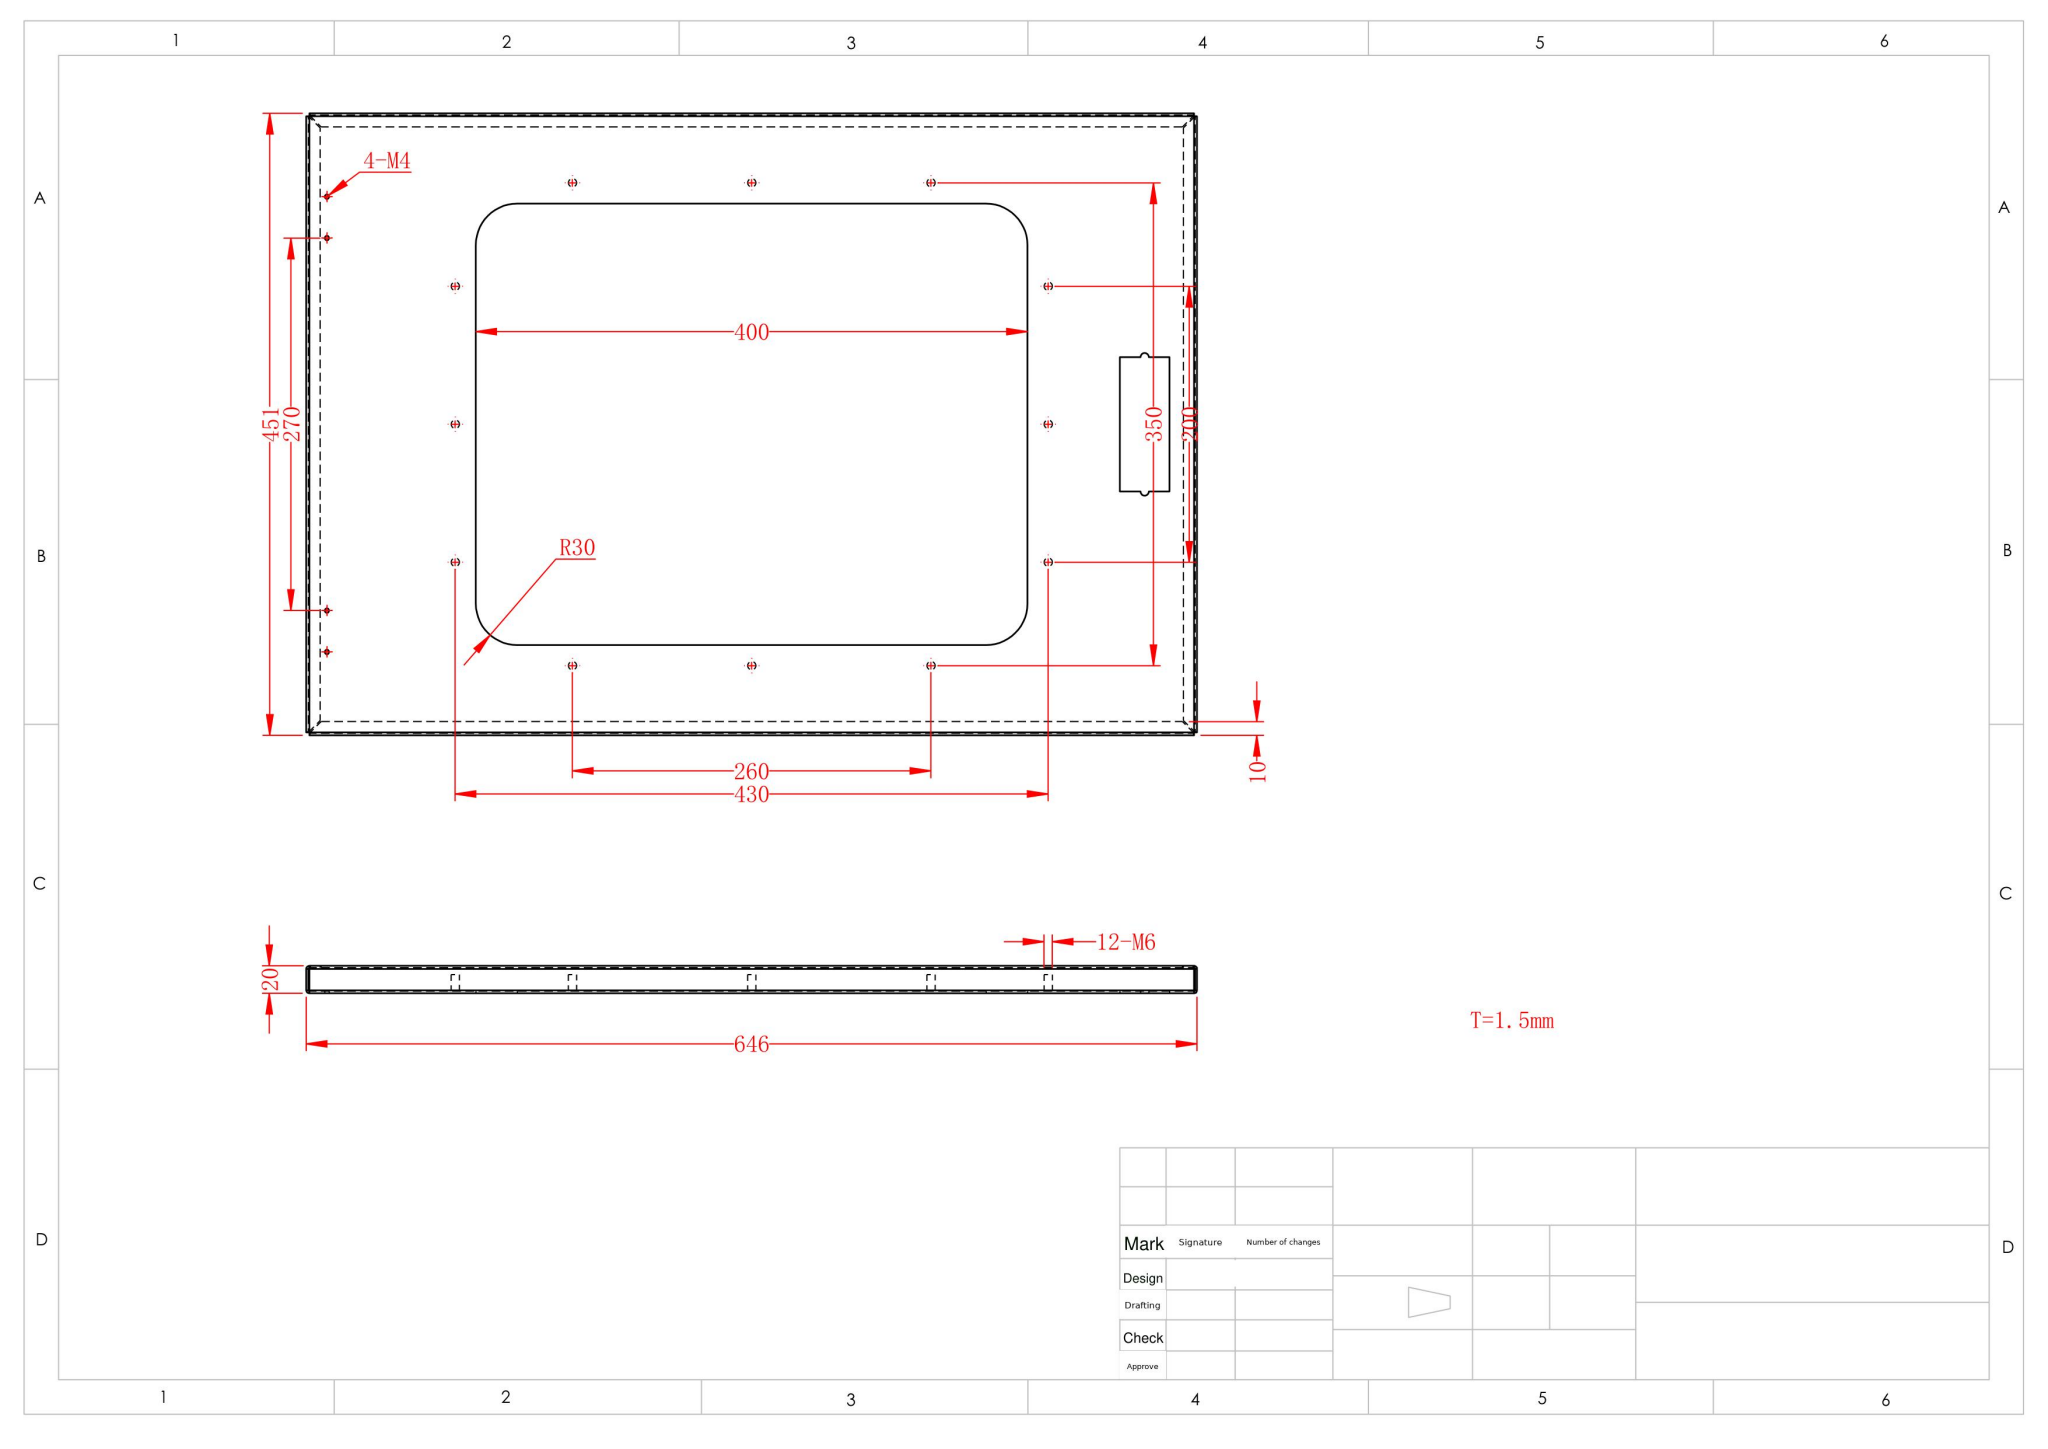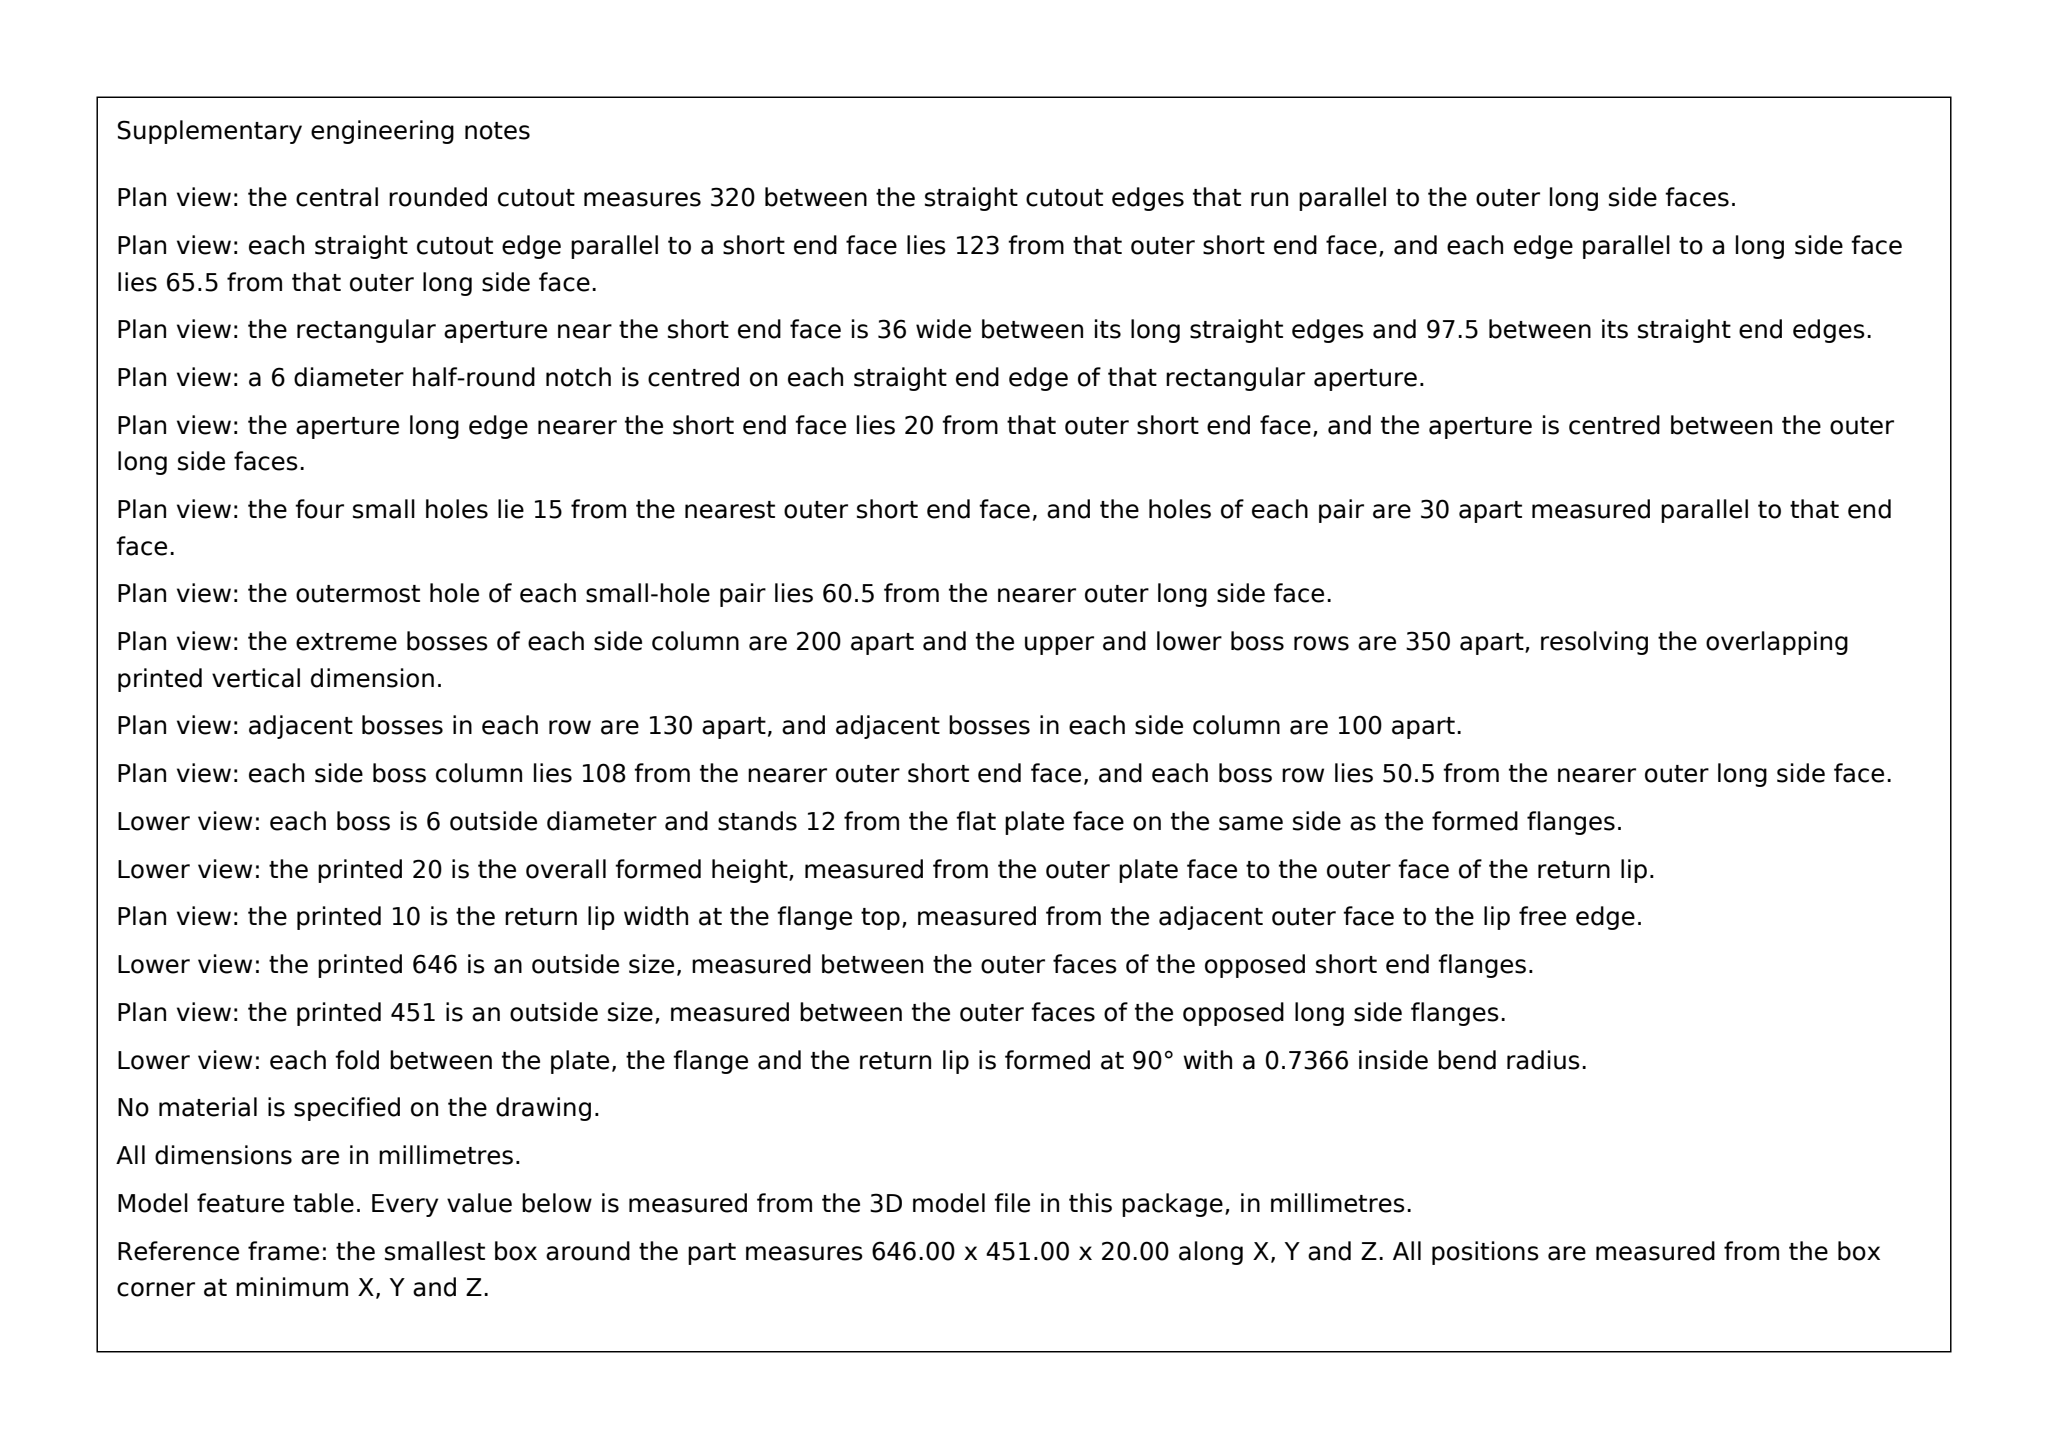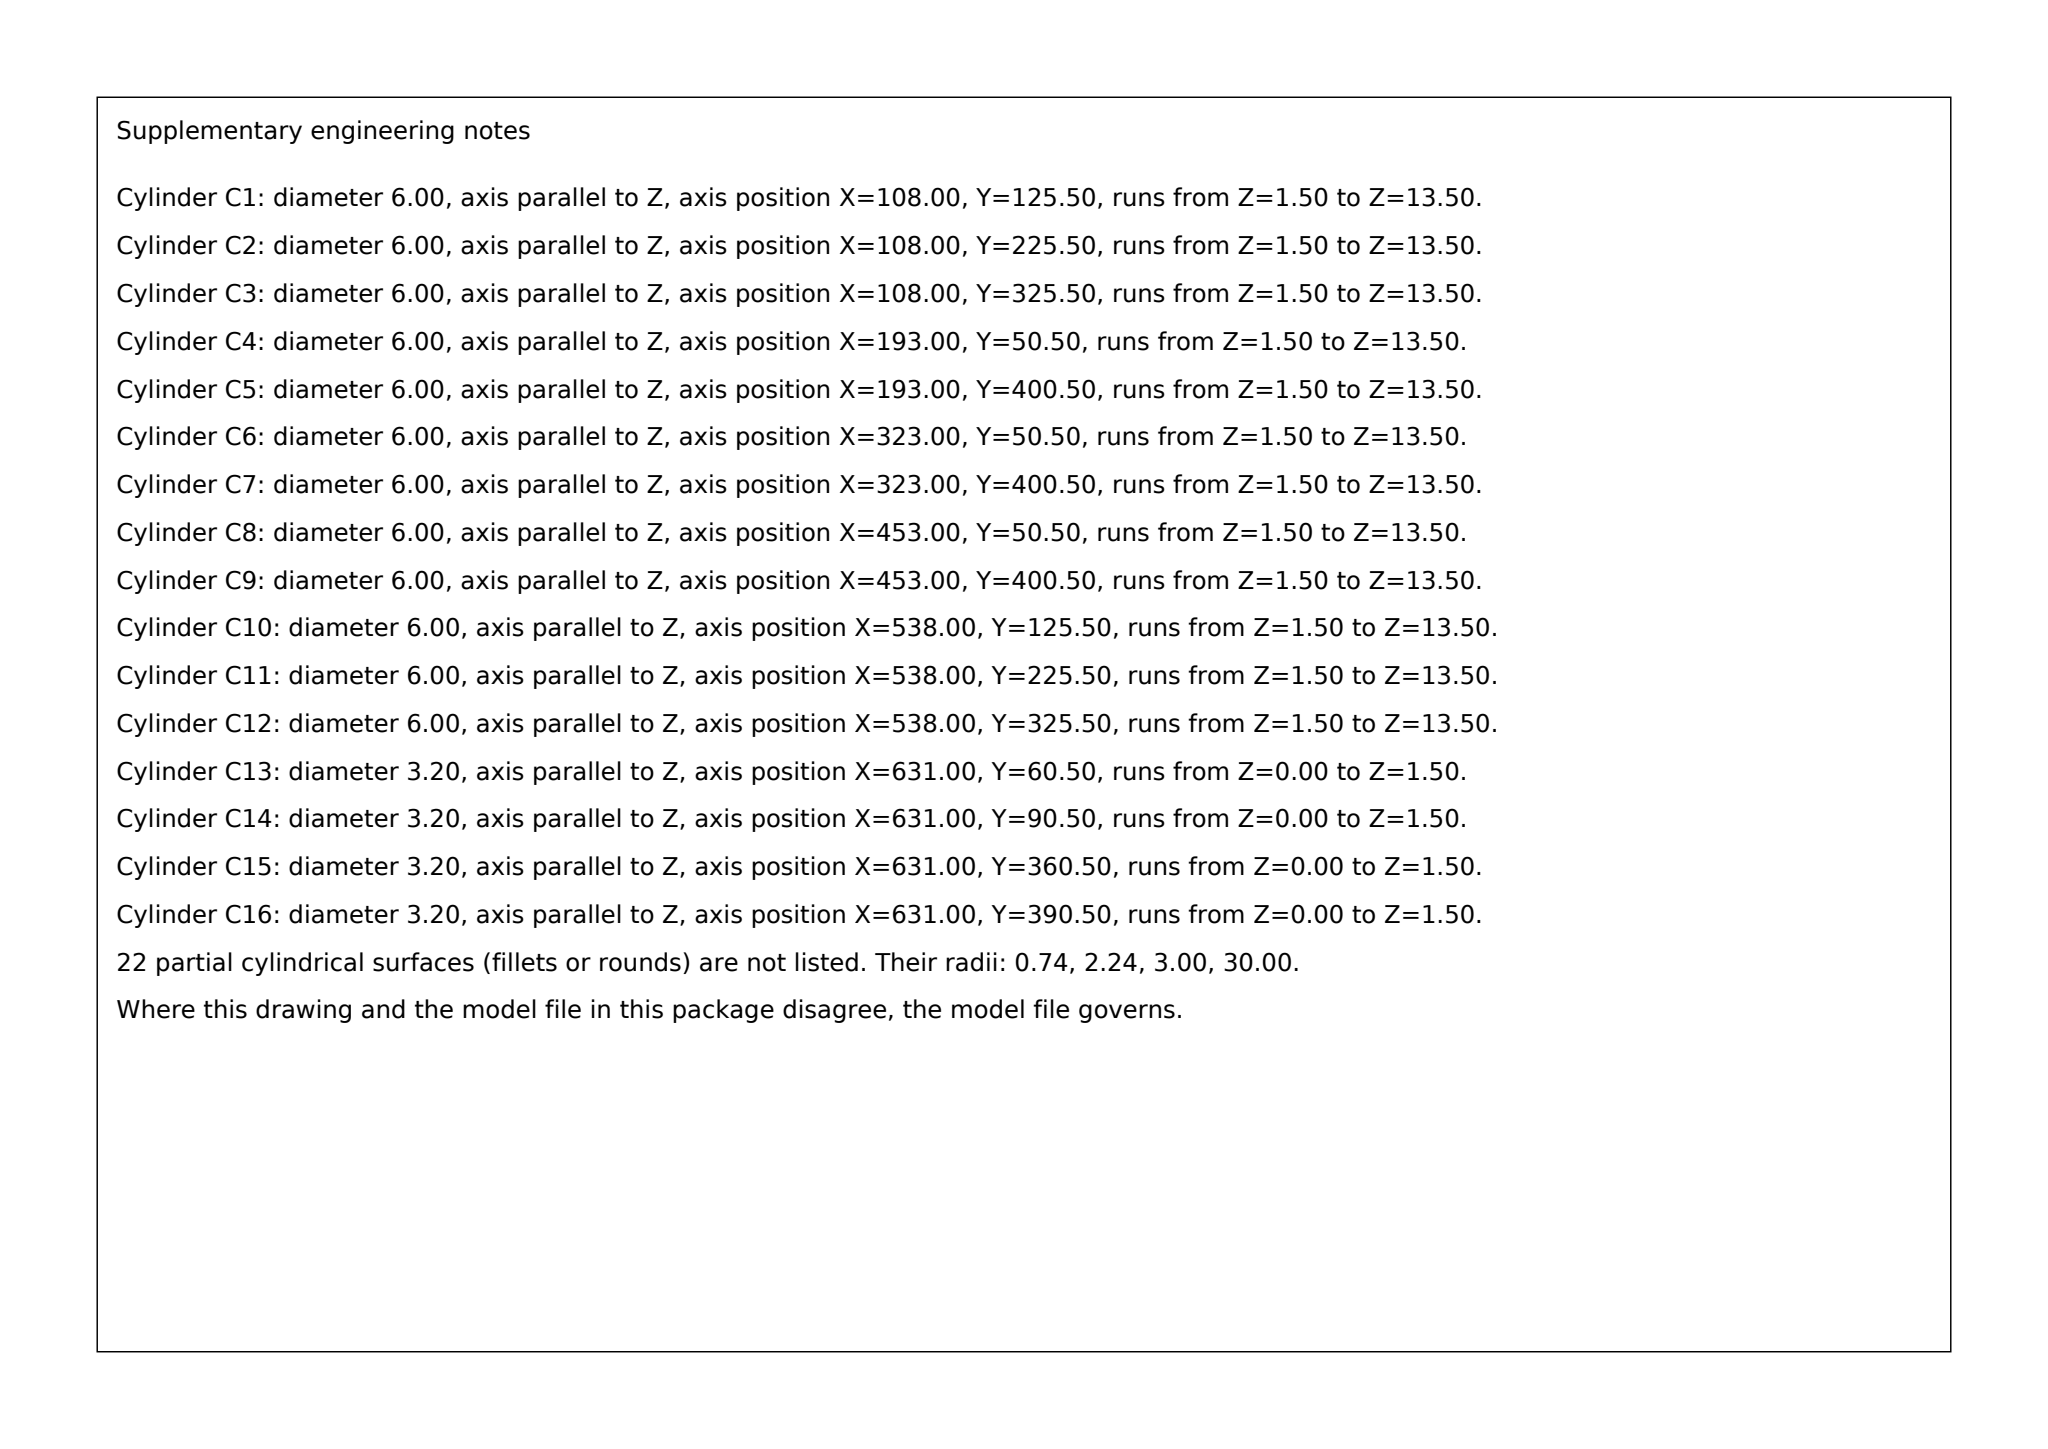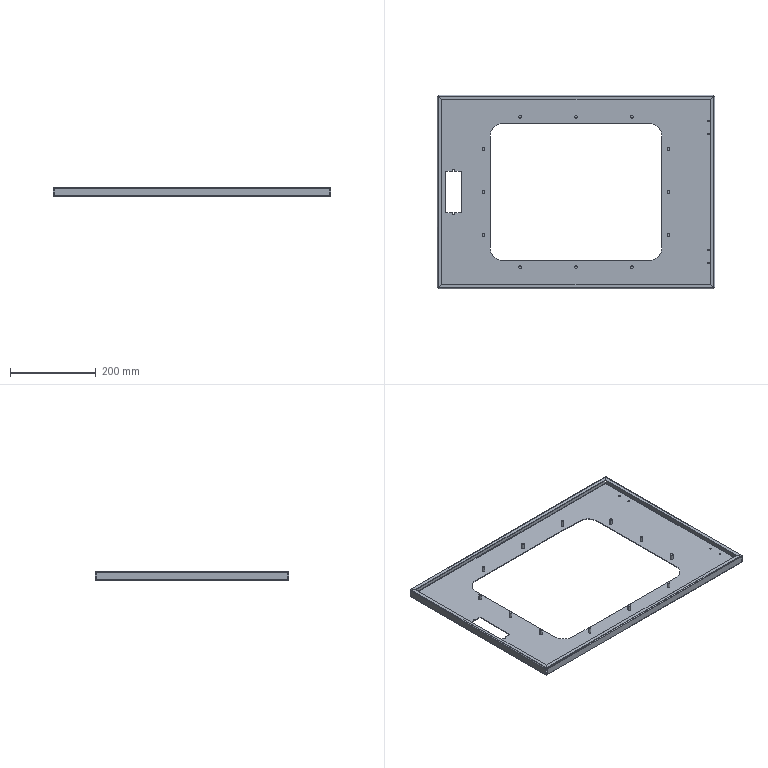Part | SolidWorks | mm | 1 solid | 130 faces | box 646 x 451 x 20 mm | volume 328400 mm3 | plane 60 | cylinder 54 | spline 16 | commonest cylinder face diameters 6 x26 3.2 x8 4.473 x8 1.473 x8 60 x4
Drawing notes:
ALL BEND RAD R0.75 INSIDE / R2.24 OUTSIDE (T=1.5) | from the solid: Bend cylinders dia 1.473 (R0.736 inner) and dia 4.473 (R2.236 outer) on all 90° flange/hem edges, T=1.5